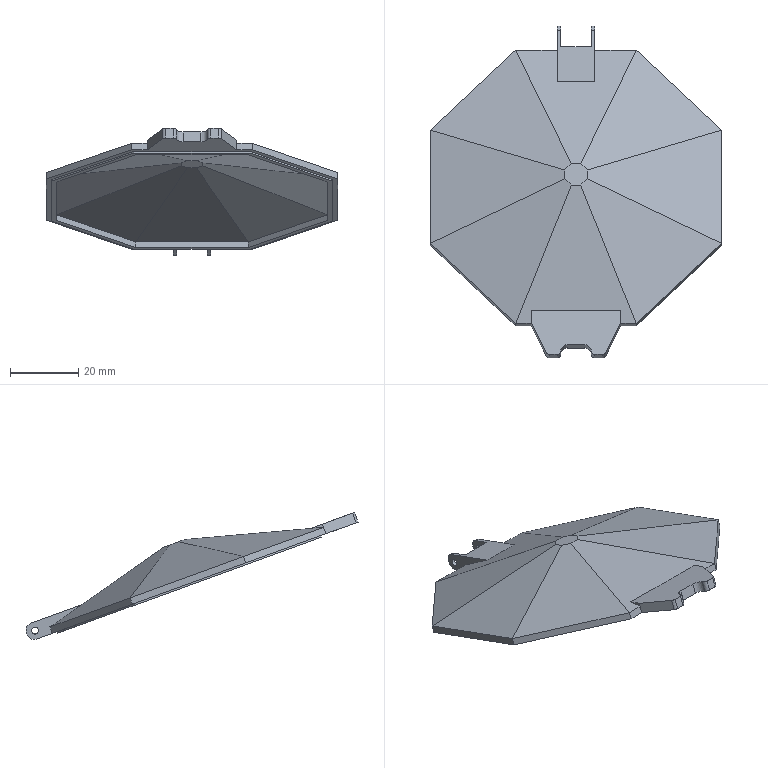Component | NX | MODEL26 | 1 solid | 74 faces | volume 11031 mm3 | plane 62 | cylinder 12 | commonest cylinder face diameters 2 x6 4 x6